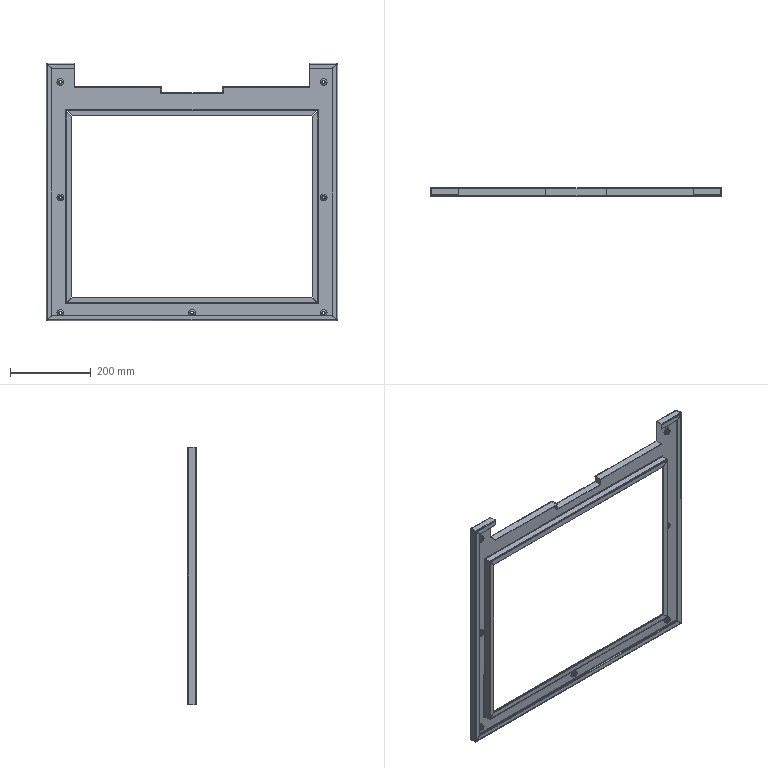Component | SolidWorks | 01-11FrontGuardPlate-1 | 1 solid | 364 faces | volume 402657 mm3 | plane 150 | cylinder 98 | spline 60 | torus 56 | commonest cylinder face diameters 4.473 x15 1.473 x15 15 x14 12 x14 6.5 x14 2 x12 5 x8 7 x6 | material SPCC